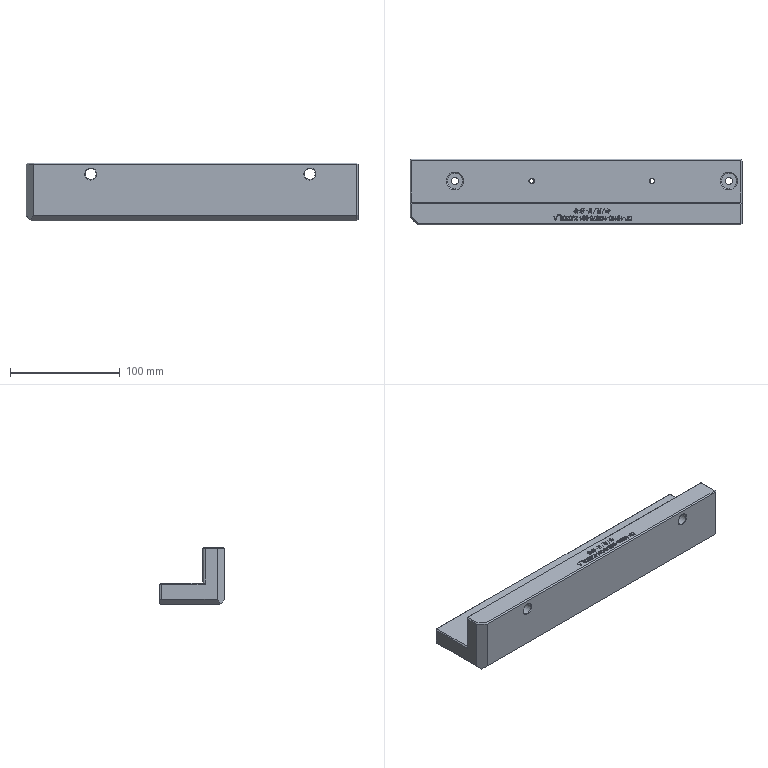CAM job | NX | mm | 3-axis | 5 set-ups | 52 operations | part box 303 x 60 x 52.8
set-up 1
1. Face Milling | Mill Mill5 E50R0.8 | FACE_MILLING_1 | path 1733.6 mm | 2.037 min
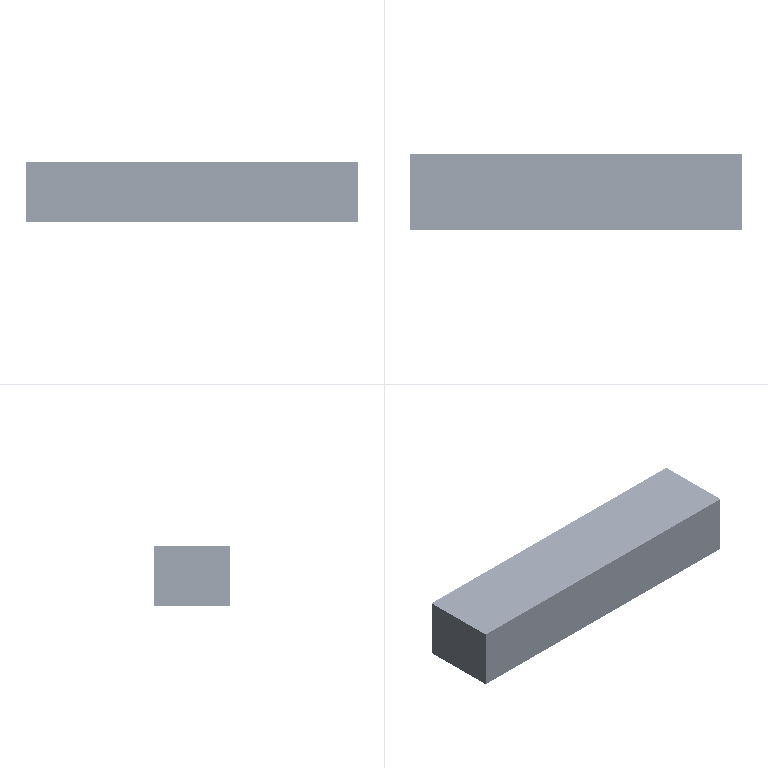2. Planar Roughing | Mill Mill5 LX-D12 | PLANAR_ROUGHING_2 | path 55810.726 mm | 13.751 min
3. Planar Milling | Mill Mill5 LX-D12J | PLANAR_MILLING_3 | path 9629.659 mm | 4.77 min
set-up 2
4. Face Milling | Mill Mill5 E50R0.8 | FACE_MILLING_4 | path 2580.133 mm | 1.216 min
5. Planar Roughing | Mill Mill5 LX-D12 | PLANAR_ROUGHING_5 | path 20187.127 mm | 4.504 min
6. Drilling | Mill MillChamfer DXZ-D10A90 | DRILLING_6 | path 204 mm | 0.0996 min
7. Drilling | Mill MillChamfer DXZ-D10A90 | DRILLING_7 | path 344 mm | 0.1136 min
8. Drilling | Drill DrillStandard ZT-D6.3 | DRILLING_8 | path 798.069 mm | 1.029 min
9. Drilling | Drill DrillStandard ZT-D3.8 | DRILLING_9 | path 1350.798 mm | 0.9453 min
10. Cylinder Milling | Mill Mill5 LX-D6 | CYLINDER_MILLING_10 | path 980.438 mm | 0.9708 min
11. Face Milling | Mill Mill5 E50R0.8 | FACE_MILLING_11 | path 842.667 mm | 1.003 min
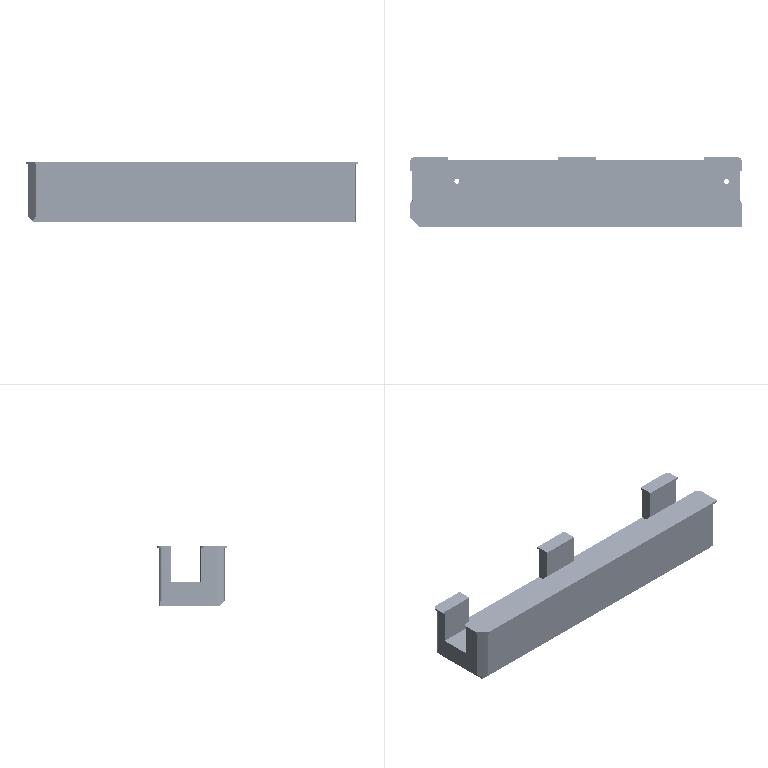12. Cylinder Milling | Mill Mill5 LX-D6J | CYLINDER_MILLING_12 | path 671.805 mm | 1.148 min
13. Cylinder Milling | Mill Mill5 LX-D4J | CYLINDER_MILLING_13 | path 780.196 mm | 1.094 min
14. Cylinder Milling | Mill Mill5 LX-D3J | CYLINDER_MILLING_14 | path 416.84 mm | 0.4 min
15. Planar Milling | Mill Mill5 LX-D12J | PLANAR_MILLING_15 | path 2528.482 mm | 2.899 min
16. Volume Based 2.5D Milling | Mill MillChamfer DJ-D10A90 | VOLUME_BASED_2.5D_MILLING_16 | path 264.24 mm | 0.09611 min
17. Volume Based 2.5D Milling | Mill MillChamfer DJ-D10A90 | VOLUME_BASED_2.5D_MILLING_17 | path 379.779 mm | 0.07509 min
18. Volume Based 2.5D Milling | Mill MillChamfer DJ-D10A90 | VOLUME_BASED_2.5D_MILLING_18 | path 411.754 mm | 0.4583 min
19. Z-Level Milling | Mill Mill5 YB-D10R1 | Z-LEVEL_MILLING_19 | path 3286.927 mm | 1.623 min
20. Z-Level Milling | Mill Mill5 YB-D10R1 | Z-LEVEL_MILLING_20 | path 17486.386 mm | 8.607 min
21. Planar Milling | Mill Mill5 LX-D12J | PLANAR_MILLING_21 | path 8144.916 mm | 4.048 min
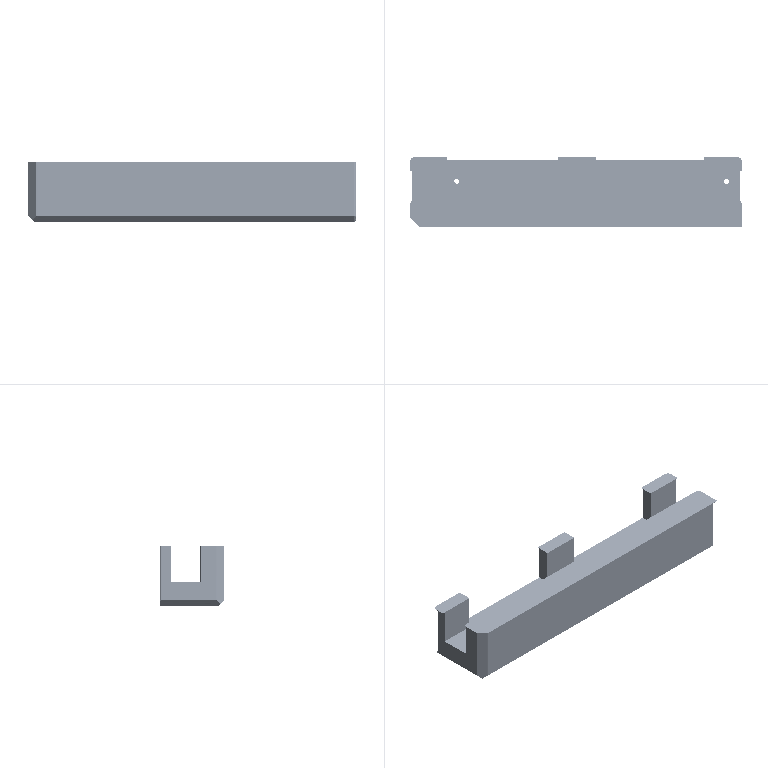set-up 3
22. Face Milling | Mill Mill5 E50R0.8 | FACE_MILLING_22 | path 2580.133 mm | 1.216 min
23. Cavity Milling | Mill Mill5 LX-D12 | CAVITY_MILLING_23 | path 71725.084 mm | 15.066 min
24. Cylinder Milling | Mill Mill5 LX-D8 | CYLINDER_MILLING_24 | path 1231.419 mm | 0.9904 min
25. Volume Based 2.5D Milling | Mill Mill5 LX-D12J | VOLUME_BASED_2.5D_MILLING_25 | path 1072.58 mm | 1.23 min
26. Volume Based 2.5D Milling | Mill Mill5 LX-D12J | VOLUME_BASED_2.5D_MILLING_26 | path 2048.719 mm | 2.446 min
27. Volume Based 2.5D Milling | Mill Mill5 LX-D12J | VOLUME_BASED_2.5D_MILLING_27 | path 1882.003 mm | 1.336 min
28. Cylinder Milling | Mill Mill5 LX-D8J | CYLINDER_MILLING_28 | path 923.195 mm | 1.162 min
29. Volume Based 2.5D Milling | Mill MillChamfer DJ-D10A90 | VOLUME_BASED_2.5D_MILLING_29 | path 706.46 mm | 0.8267 min
30. Volume Based 2.5D Milling | Mill MillChamfer DJ-D10A90 | VOLUME_BASED_2.5D_MILLING_30 | path 571.032 mm | 0.1556 min
31. Drilling | Mill MillChamfer DJ-D10A90 | DRILLING_31 | path 341.2 mm | 0.1077 min
32. Volume Based 2.5D Milling | Mill MillChamfer DJ-D4A90 | VOLUME_BASED_2.5D_MILLING_32 | path 1300.31 mm | 1.013 min
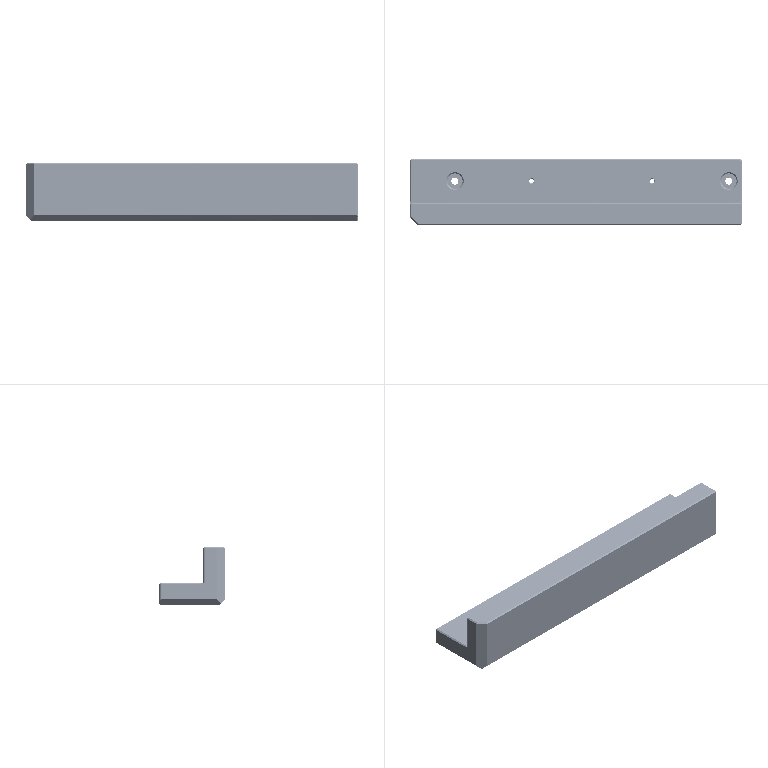33. Planar Text | Mill Mill5 KZ-D0.5R0.25 | PLANAR_TEXT_33 | path 21094.199 mm | 5.329 min
34. Planar Milling | Mill Mill5 LX-D12J | PLANAR_MILLING_34 | path 8174.537 mm | 4.059 min
set-up 4
35. Cavity Milling | Mill Mill5 LX-D8 | CAVITY_MILLING_35 | path 6107.07 mm | 4.187 min
36. Cylinder Milling | Mill Mill5 LX-D8 | CYLINDER_MILLING_36 | path 850.489 mm | 0.4993 min
37. Cylinder Milling | Mill Mill5 LX-D8J | CYLINDER_MILLING_37 | path 1053.924 mm | 1.584 min
38. Planar Milling | Mill Mill5 LX-D8J | PLANAR_MILLING_38 | path 578.753 mm | 0.1895 min
39. Cylinder Milling | Mill Mill5 LX-D8J | CYLINDER_MILLING_39 | path 685.386 mm | 0.5381 min
40. Cavity Milling | Mill Mill5 LX-D4J | CAVITY_MILLING_40 | path 1392.762 mm | 0.3674 min
41. Volume Based 2.5D Milling | Mill MillChamfer DJ-D10A90 | VOLUME_BASED_2.5D_MILLING_41 | path 581.957 mm | 0.2222 min
42. Volume Based 2.5D Milling | Mill MillChamfer DJ-D10A90 | VOLUME_BASED_2.5D_MILLING_42 | path 532.239 mm | 0.1229 min
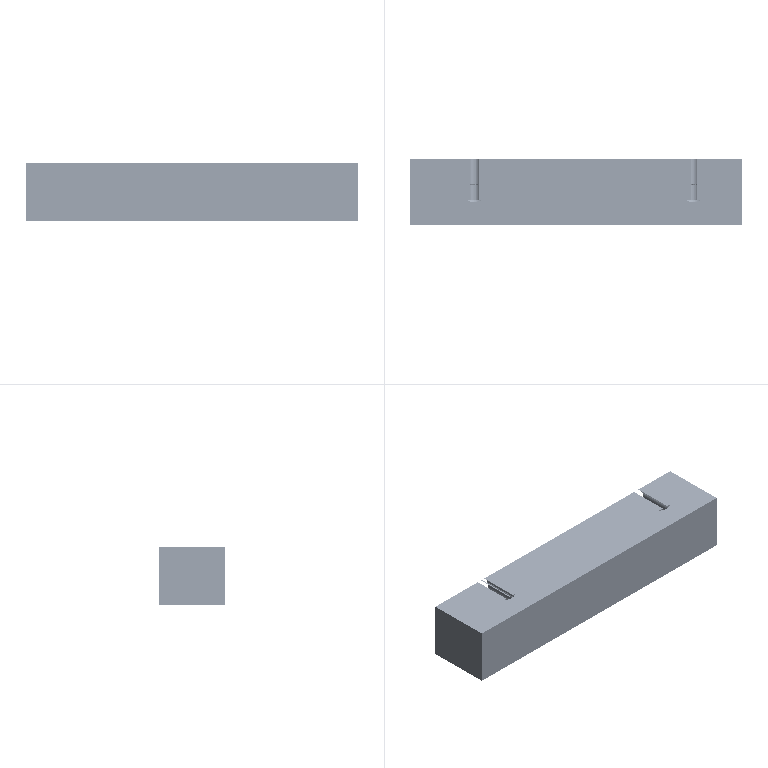43. Drilling | Mill MillChamfer DXZ-D4A90 | DRILLING_43 | path 137 mm | 0.0533 min
44. Drilling | Mill MillChamfer DXZ-D4A90 | DRILLING_44 | path 137 mm | 0.0533 min
45. Drilling | Drill DrillStandard ZT-D3.3 | DRILLING_45 | path 429.803 mm | 0.2531 min
46. Drilling | Drill DrillStandard ZT-D3.3 | DRILLING_46 | path 429.803 mm | 0.2531 min
47. Volume Based 2.5D Milling | Mill MillChamfer DJ-D4A90 | VOLUME_BASED_2.5D_MILLING_47 | path 598.858 mm | 0.2109 min
48. Thread Milling | Drill DrillThreadMill M4X0.7-D3.15 | THREAD_MILLING_48 | path 254.154 mm | 0.1983 min
49. Thread Milling | Drill DrillThreadMill M4X0.7-D3.15 | THREAD_MILLING_49 | path 254.154 mm | 0.1983 min
50. Thread Milling | Drill DrillThreadMill M4X0.7-D3.15 | THREAD_MILLING_50 | path 183.351 mm | 0.09519 min
51. Thread Milling | Drill DrillThreadMill M4X0.7-D3.15 | THREAD_MILLING_51 | path 183.351 mm | 0.09519 min
set-up 5
52. Volume Based 2.5D Milling | Mill MillChamfer DJ-D10A90 | VOLUME_BASED_2.5D_MILLING_52 | path 350.924 mm | 0.1048 min